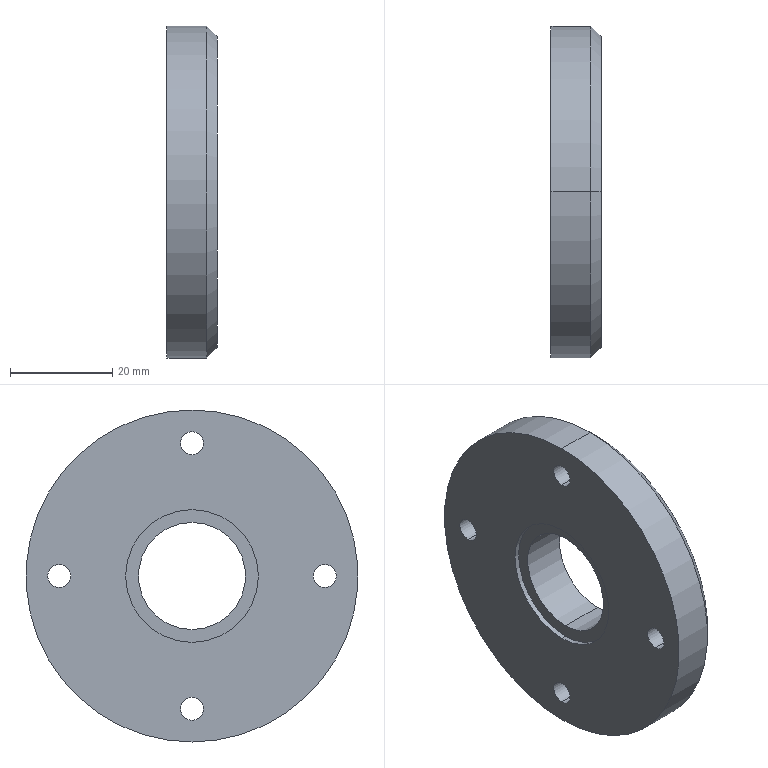Component | SolidWorks | ChainPartBearingInnerEndCap-1 | 1 solid | 19 faces | box 9.8 x 65 x 65 mm | volume 27917 mm3 | cylinder 14 | plane 3 | cone 2 | commonest cylinder face diameters 4.5 x8 26 x2 65 x2 21 x2
build123d program:
from build123d import *

# Parameters (mm, degrees)
CHAMFER1_SIZE              = 2
F_4_5_4_5_DIAMETER_HOLE1_D = 4.5


with BuildPart() as part:
    # Sketch1 → Revolve1 (revolve)
    with BuildSketch(Plane.XY, mode=Mode.PRIVATE) as revolve1_sk:
        Polygon((10.5, 0), (32.5, 0), (32.5, 9.8), (13, 9.8), (13, 8.8), (10.5, 8.8), align=None)
    revolve(revolve1_sk.sketch.rotate(Axis((0, 0, 0), (0, 1, 0)), 90), axis=Axis((0, 0, 0), (0, 1, 0)))

    # Chamfer1
    chamfer1_edges = [part.edges().sort_by_distance(p)[0] for p in [
        (0, 0, 32.5),
    ]]
    chamfer(chamfer1_edges, length=CHAMFER1_SIZE)

    # 4.5 _4.5_ Diameter Hole1 (through all)
    with Locations(Plane(origin=(0, 0, 0), x_dir=(-1, 0, 0), z_dir=(0, -1, 0))):
        with Locations((0, -26), (26, 0), (0, 26), (-26, 0)):
            Hole(F_4_5_4_5_DIAMETER_HOLE1_D / 2)


solid = part.part

# Placed as in the assembly
solid = solid.moved(Location((145.437, -2.563, -35.304), (0, 0, 90)))